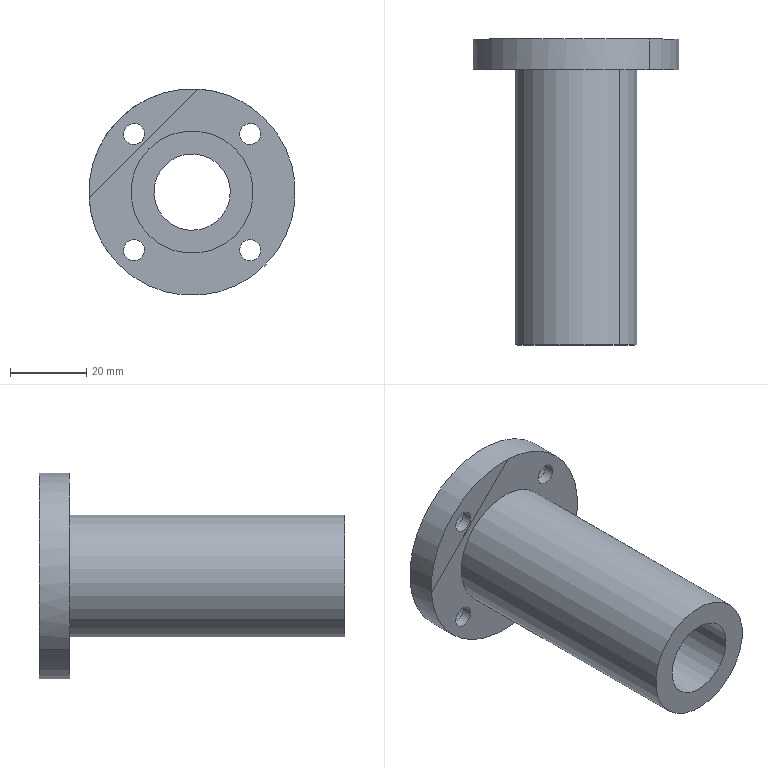Component | SolidWorks | LinearBearing20mmStandardRoundFlangeDoubleLinerTypeLMF20LUU-1 | 1 solid | 31 faces | box 54 x 80 x 54 mm | volume 49314 mm3 | cylinder 22 | plane 9 | commonest cylinder face diameters 9.5 x8 5.5 x8 20 x2 32 x2 54 x2
build123d program:
from build123d import *

# Parameters (mm, degrees)
SKETCH1_R                                       = 27
BOSS_EXTRUDE1_DEPTH                             = 8
SKETCH2_R                                       = 16
BOSS_EXTRUDE2_DEPTH                             = 72
SKETCH3_R                                       = 10
CUT_EXTRUDE1_DEPTH                              = 89.645
M5_HEX_SOCKET_HEAD_CAP_SCREW_CBORE1_D           = 5.5
M5_HEX_SOCKET_HEAD_CAP_SCREW_CBORE1_CBORE_D     = 9.5
M5_HEX_SOCKET_HEAD_CAP_SCREW_CBORE1_CBORE_DEPTH = 5.4
CIRPATTERN1_COUNT                               = 4
SKETCH7_W                                       = 60.924
SKETCH7_H                                       = 19.438
CUT_EXTRUDE2_DEPTH                              = 0.01


with BuildPart() as part:
    # Sketch1 → Boss-Extrude1 (new body)
    with BuildSketch(Plane.XY):
        Circle(SKETCH1_R)
    extrude(amount=BOSS_EXTRUDE1_DEPTH)

    # Sketch2 → Boss-Extrude2 (add)
    with BuildSketch(Plane.XY.offset(8)):
        Circle(SKETCH2_R)
    extrude(amount=BOSS_EXTRUDE2_DEPTH)

    # Sketch3 → Cut-Extrude1 (cut, through all)
    with BuildSketch(Plane(origin=(0, 0, 0), x_dir=(-1, 0, 0), z_dir=(0, 0, -1))):
        Circle(SKETCH3_R)
    extrude(amount=-CUT_EXTRUDE1_DEPTH, mode=Mode.SUBTRACT)

    # M5 Hex Socket Head Cap Screw CBORE1 (through all)
    with Locations(Plane(origin=(0, 0, 0), x_dir=(-1, 0, 0), z_dir=(0, 0, -1))):
        with Locations((0, -21.5)):
            m5_hex_socket_head_cap_screw_cbore1 = CounterBoreHole(M5_HEX_SOCKET_HEAD_CAP_SCREW_CBORE1_D / 2, M5_HEX_SOCKET_HEAD_CAP_SCREW_CBORE1_CBORE_D / 2, M5_HEX_SOCKET_HEAD_CAP_SCREW_CBORE1_CBORE_DEPTH)

    # CirPattern1: M5 Hex Socket Head Cap Screw CBORE1 ×4 about axis
    cirpattern1_axis = Axis((0, 0, 0), (0, 0, 1))
    for i in range(1, CIRPATTERN1_COUNT):
        add(m5_hex_socket_head_cap_screw_cbore1.rotate(cirpattern1_axis, i * 360 / CIRPATTERN1_COUNT), mode=Mode.SUBTRACT)

    # Sketch7 → Cut-Extrude2 (cut)
    with BuildSketch(Plane.XY.offset(8)):
        with Locations((-1.946, -27.719)):
            Rectangle(SKETCH7_W, SKETCH7_H)
    extrude(amount=-CUT_EXTRUDE2_DEPTH, mode=Mode.SUBTRACT)


solid = part.part

# Placed as in the assembly
solid = solid.moved(Location((-641.612, -154.873, 2398.4), (90, 0, -135)))
STEP:
#1=COLOUR_RGB('',0.7922,0.8196,0.9333);
#2=FILL_AREA_STYLE_COLOUR('',#1);
#3=FILL_AREA_STYLE('',(#2));
#4=SURFACE_STYLE_FILL_AREA(#3);
#5=SURFACE_SIDE_STYLE('',(#4));
#6=SURFACE_STYLE_USAGE(.BOTH.,#5);
#7=PRESENTATION_STYLE_ASSIGNMENT((#6));
#8=CARTESIAN_POINT('',(-25.991,-6.31,93.694));
#9=VERTEX_POINT('',#8);
#10=CARTESIAN_POINT('',(-25.727,-6.31,93.959));
#11=VERTEX_POINT('',#10);
#12=CARTESIAN_POINT('',(-25.859,-6.31,93.827));
#13=DIRECTION('',(-0.,1.,-0.));
#14=DIRECTION('',(0.7071,0.,0.7071));
#15=AXIS2_PLACEMENT_3D('',#12,#13,#14);
#16=CIRCLE('',#15,0.187);
#17=EDGE_CURVE('',#9,#11,#16,.T.);
#18=ORIENTED_EDGE('',*,*,#17,.F.);
#19=CARTESIAN_POINT('',(-25.991,-6.097,93.694));
#20=VERTEX_POINT('',#19);
#21=CARTESIAN_POINT('',(-25.991,-6.097,93.694));
#22=DIRECTION('',(-0.,1.,-0.));
#23=VECTOR('',#22,39.37);
#24=LINE('',#21,#23);
#25=EDGE_CURVE('',#9,#20,#24,.T.);
#26=ORIENTED_EDGE('',*,*,#25,.T.);
#27=CARTESIAN_POINT('',(-25.727,-6.097,93.959));
#28=VERTEX_POINT('',#27);
#29=CARTESIAN_POINT('',(-25.859,-6.097,93.827));
#30=DIRECTION('',(-0.,1.,-0.));
#31=DIRECTION('',(0.7071,0.,0.7071));
#32=AXIS2_PLACEMENT_3D('',#29,#30,#31);
#33=CIRCLE('',#32,0.187);
#34=EDGE_CURVE('',#20,#28,#33,.T.);
#35=ORIENTED_EDGE('',*,*,#34,.T.);
#36=CARTESIAN_POINT('',(-25.727,-6.097,93.959));
#37=DIRECTION('',(-0.,1.,-0.));
#38=VECTOR('',#37,39.37);
#39=LINE('',#36,#38);
#40=EDGE_CURVE('',#11,#28,#39,.T.);
#41=ORIENTED_EDGE('',*,*,#40,.F.);
#42=EDGE_LOOP('',(#18,#26,#35,#41));
#43=FACE_OUTER_BOUND('',#42,.T.);
#44=CARTESIAN_POINT('',(-25.859,-6.097,93.827));
#45=DIRECTION('',(-0.,1.,-0.));
#46=DIRECTION('',(0.7071,0.,0.7071));
#47=AXIS2_PLACEMENT_3D('',#44,#45,#46);
#48=CYLINDRICAL_SURFACE('',#47,0.187);
#49=ADVANCED_FACE('',(#43),#48,.F.);
#50=CARTESIAN_POINT('',(-25.782,-6.412,93.903));
#51=VERTEX_POINT('',#50);
#52=CARTESIAN_POINT('',(-25.935,-6.412,93.75));
#53=VERTEX_POINT('',#52);
#54=CARTESIAN_POINT('',(-25.859,-6.412,93.827));
#55=DIRECTION('',(0.,-1.,0.));
#56=DIRECTION('',(-0.7071,0.,-0.7071));
#57=AXIS2_PLACEMENT_3D('',#54,#55,#56);
#58=CIRCLE('',#57,0.1083);
#59=EDGE_CURVE('',#51,#53,#58,.T.);
#60=ORIENTED_EDGE('',*,*,#59,.T.);
#61=CARTESIAN_POINT('',(-25.935,-6.31,93.75));
#62=VERTEX_POINT('',#61);
#63=CARTESIAN_POINT('',(-25.935,-6.097,93.75));
#64=DIRECTION('',(-0.,1.,-0.));
#65=VECTOR('',#64,39.37);
#66=LINE('',#63,#65);
#67=EDGE_CURVE('',#53,#62,#66,.T.);
#68=ORIENTED_EDGE('',*,*,#67,.T.);
#69=CARTESIAN_POINT('',(-25.782,-6.31,93.903));
#70=VERTEX_POINT('',#69);
#71=CARTESIAN_POINT('',(-25.859,-6.31,93.827));
#72=DIRECTION('',(-0.,1.,-0.));
#73=DIRECTION('',(0.7071,0.,0.7071));
#74=AXIS2_PLACEMENT_3D('',#71,#72,#73);
#75=CIRCLE('',#74,0.1083);
#76=EDGE_CURVE('',#62,#70,#75,.T.);
#77=ORIENTED_EDGE('',*,*,#76,.T.);
#78=CARTESIAN_POINT('',(-25.782,-6.097,93.903));
#79=DIRECTION('',(-0.,1.,-0.));
#80=VECTOR('',#79,39.37);
#81=LINE('',#78,#80);
#82=EDGE_CURVE('',#51,#70,#81,.T.);
#83=ORIENTED_EDGE('',*,*,#82,.F.);
#84=EDGE_LOOP('',(#60,#68,#77,#83));
#85=FACE_OUTER_BOUND('',#84,.T.);
#86=CARTESIAN_POINT('',(-25.859,-6.097,93.827));
#87=DIRECTION('',(-0.,1.,-0.));
#88=DIRECTION('',(0.7071,0.,0.7071));
#89=AXIS2_PLACEMENT_3D('',#86,#87,#88);
#90=CYLINDRICAL_SURFACE('',#89,0.1083);
#91=ADVANCED_FACE('',(#85),#90,.F.);
#92=CARTESIAN_POINT('',(-24.794,-6.31,93.694));
#93=VERTEX_POINT('',#92);
#94=CARTESIAN_POINT('',(-24.53,-6.31,93.959));
#95=VERTEX_POINT('',#94);
#96=CARTESIAN_POINT('',(-24.662,-6.31,93.827));
#97=DIRECTION('',(-0.,1.,-0.));
#98=DIRECTION('',(0.7071,0.,0.7071));
#99=AXIS2_PLACEMENT_3D('',#96,#97,#98);
#100=CIRCLE('',#99,0.187);
#101=EDGE_CURVE('',#93,#95,#100,.T.);
#102=ORIENTED_EDGE('',*,*,#101,.F.);
#103=CARTESIAN_POINT('',(-24.794,-6.097,93.694));
#104=VERTEX_POINT('',#103);
#105=CARTESIAN_POINT('',(-24.794,-6.097,93.694));
#106=DIRECTION('',(-0.,1.,-0.));
#107=VECTOR('',#106,39.37);
#108=LINE('',#105,#107);
#109=EDGE_CURVE('',#93,#104,#108,.T.);
#110=ORIENTED_EDGE('',*,*,#109,.T.);
#111=CARTESIAN_POINT('',(-24.53,-6.097,93.959));
#112=VERTEX_POINT('',#111);
#113=CARTESIAN_POINT('',(-24.662,-6.097,93.827));
#114=DIRECTION('',(-0.,1.,-0.));
#115=DIRECTION('',(0.7071,0.,0.7071));
#116=AXIS2_PLACEMENT_3D('',#113,#114,#115);
#117=CIRCLE('',#116,0.187);
#118=EDGE_CURVE('',#104,#112,#117,.T.);
#119=ORIENTED_EDGE('',*,*,#118,.T.);
#120=CARTESIAN_POINT('',(-24.53,-6.097,93.959));
#121=DIRECTION('',(-0.,1.,-0.));
#122=VECTOR('',#121,39.37);
#123=LINE('',#120,#122);
#124=EDGE_CURVE('',#95,#112,#123,.T.);
#125=ORIENTED_EDGE('',*,*,#124,.F.);
#126=EDGE_LOOP('',(#102,#110,#119,#125));
#127=FACE_OUTER_BOUND('',#126,.T.);
#128=CARTESIAN_POINT('',(-24.662,-6.097,93.827));
#129=DIRECTION('',(-0.,1.,-0.));
#130=DIRECTION('',(0.7071,0.,0.7071));
#131=AXIS2_PLACEMENT_3D('',#128,#129,#130);
#132=CYLINDRICAL_SURFACE('',#131,0.187);
#133=ADVANCED_FACE('',(#127),#132,.F.);
#134=CARTESIAN_POINT('',(-24.585,-6.412,93.903));
#135=VERTEX_POINT('',#134);
#136=CARTESIAN_POINT('',(-24.738,-6.412,93.75));
#137=VERTEX_POINT('',#136);
#138=CARTESIAN_POINT('',(-24.662,-6.412,93.827));
#139=DIRECTION('',(0.,-1.,0.));
#140=DIRECTION('',(-0.7071,0.,-0.7071));
#141=AXIS2_PLACEMENT_3D('',#138,#139,#140);
#142=CIRCLE('',#141,0.1083);
#143=EDGE_CURVE('',#135,#137,#142,.T.);
#144=ORIENTED_EDGE('',*,*,#143,.T.);
#145=CARTESIAN_POINT('',(-24.738,-6.31,93.75));
#146=VERTEX_POINT('',#145);
#147=CARTESIAN_POINT('',(-24.738,-6.097,93.75));
#148=DIRECTION('',(-0.,1.,-0.));
#149=VECTOR('',#148,39.37);
#150=LINE('',#147,#149);
#151=EDGE_CURVE('',#137,#146,#150,.T.);
#152=ORIENTED_EDGE('',*,*,#151,.T.);
#153=CARTESIAN_POINT('',(-24.585,-6.31,93.903));
#154=VERTEX_POINT('',#153);
#155=CARTESIAN_POINT('',(-24.662,-6.31,93.827));
#156=DIRECTION('',(-0.,1.,-0.));
#157=DIRECTION('',(0.7071,0.,0.7071));
#158=AXIS2_PLACEMENT_3D('',#155,#156,#157);
#159=CIRCLE('',#158,0.1083);
#160=EDGE_CURVE('',#146,#154,#159,.T.);
#161=ORIENTED_EDGE('',*,*,#160,.T.);
#162=CARTESIAN_POINT('',(-24.585,-6.097,93.903));
#163=DIRECTION('',(-0.,1.,-0.));
#164=VECTOR('',#163,39.37);
#165=LINE('',#162,#164);
#166=EDGE_CURVE('',#135,#154,#165,.T.);
#167=ORIENTED_EDGE('',*,*,#166,.F.);
#168=EDGE_LOOP('',(#144,#152,#161,#167));
#169=FACE_OUTER_BOUND('',#168,.T.);
#170=CARTESIAN_POINT('',(-24.662,-6.097,93.827));
#171=DIRECTION('',(-0.,1.,-0.));
#172=DIRECTION('',(0.7071,0.,0.7071));
#173=AXIS2_PLACEMENT_3D('',#170,#171,#172);
#174=CYLINDRICAL_SURFACE('',#173,0.1083);
#175=ADVANCED_FACE('',(#169),#174,.F.);
#176=CARTESIAN_POINT('',(-24.794,-6.31,94.891));
#177=VERTEX_POINT('',#176);
#178=CARTESIAN_POINT('',(-24.53,-6.31,95.156));
#179=VERTEX_POINT('',#178);
#180=CARTESIAN_POINT('',(-24.662,-6.31,95.024));
#181=DIRECTION('',(-0.,1.,-0.));
#182=DIRECTION('',(0.7071,0.,0.7071));
#183=AXIS2_PLACEMENT_3D('',#180,#181,#182);
#184=CIRCLE('',#183,0.187);
#185=EDGE_CURVE('',#177,#179,#184,.T.);
#186=ORIENTED_EDGE('',*,*,#185,.F.);
#187=CARTESIAN_POINT('',(-24.794,-6.097,94.891));
#188=VERTEX_POINT('',#187);
#189=CARTESIAN_POINT('',(-24.794,-6.097,94.891));
#190=DIRECTION('',(-0.,1.,-0.));
#191=VECTOR('',#190,39.37);
#192=LINE('',#189,#191);
#193=EDGE_CURVE('',#177,#188,#192,.T.);
#194=ORIENTED_EDGE('',*,*,#193,.T.);
#195=CARTESIAN_POINT('',(-24.53,-6.097,95.156));
#196=VERTEX_POINT('',#195);
#197=CARTESIAN_POINT('',(-24.662,-6.097,95.024));
#198=DIRECTION('',(-0.,1.,-0.));
#199=DIRECTION('',(0.7071,0.,0.7071));
#200=AXIS2_PLACEMENT_3D('',#197,#198,#199);
#201=CIRCLE('',#200,0.187);
#202=EDGE_CURVE('',#188,#196,#201,.T.);
#203=ORIENTED_EDGE('',*,*,#202,.T.);
#204=CARTESIAN_POINT('',(-24.53,-6.097,95.156));
#205=DIRECTION('',(-0.,1.,-0.));
#206=VECTOR('',#205,39.37);
#207=LINE('',#204,#206);
#208=EDGE_CURVE('',#179,#196,#207,.T.);
#209=ORIENTED_EDGE('',*,*,#208,.F.);
#210=EDGE_LOOP('',(#186,#194,#203,#209));
#211=FACE_OUTER_BOUND('',#210,.T.);
#212=CARTESIAN_POINT('',(-24.662,-6.097,95.024));
#213=DIRECTION('',(-0.,1.,-0.));
#214=DIRECTION('',(0.7071,0.,0.7071));
#215=AXIS2_PLACEMENT_3D('',#212,#213,#214);
#216=CYLINDRICAL_SURFACE('',#215,0.187);
#217=ADVANCED_FACE('',(#211),#216,.F.);
#218=CARTESIAN_POINT('',(-24.585,-6.412,95.1));
#219=VERTEX_POINT('',#218);
#220=CARTESIAN_POINT('',(-24.738,-6.412,94.947));
#221=VERTEX_POINT('',#220);
#222=CARTESIAN_POINT('',(-24.662,-6.412,95.024));
#223=DIRECTION('',(0.,-1.,0.));
#224=DIRECTION('',(-0.7071,0.,-0.7071));
#225=AXIS2_PLACEMENT_3D('',#222,#223,#224);
#226=CIRCLE('',#225,0.1083);
#227=EDGE_CURVE('',#219,#221,#226,.T.);
#228=ORIENTED_EDGE('',*,*,#227,.T.);
#229=CARTESIAN_POINT('',(-24.738,-6.31,94.947));
#230=VERTEX_POINT('',#229);
#231=CARTESIAN_POINT('',(-24.738,-6.097,94.947));
#232=DIRECTION('',(-0.,1.,-0.));
#233=VECTOR('',#232,39.37);
#234=LINE('',#231,#233);
#235=EDGE_CURVE('',#221,#230,#234,.T.);
#236=ORIENTED_EDGE('',*,*,#235,.T.);
#237=CARTESIAN_POINT('',(-24.585,-6.31,95.1));
#238=VERTEX_POINT('',#237);
#239=CARTESIAN_POINT('',(-24.662,-6.31,95.024));
#240=DIRECTION('',(-0.,1.,-0.));
#241=DIRECTION('',(0.7071,0.,0.7071));
#242=AXIS2_PLACEMENT_3D('',#239,#240,#241);
#243=CIRCLE('',#242,0.1083);
#244=EDGE_CURVE('',#230,#238,#243,.T.);
#245=ORIENTED_EDGE('',*,*,#244,.T.);
#246=CARTESIAN_POINT('',(-24.585,-6.097,95.1));
#247=DIRECTION('',(-0.,1.,-0.));
#248=VECTOR('',#247,39.37);
#249=LINE('',#246,#248);
#250=EDGE_CURVE('',#219,#238,#249,.T.);
#251=ORIENTED_EDGE('',*,*,#250,.F.);
#252=EDGE_LOOP('',(#228,#236,#245,#251));
#253=FACE_OUTER_BOUND('',#252,.T.);
#254=CARTESIAN_POINT('',(-24.662,-6.097,95.024));
#255=DIRECTION('',(-0.,1.,-0.));
#256=DIRECTION('',(0.7071,0.,0.7071));
#257=AXIS2_PLACEMENT_3D('',#254,#255,#256);
#258=CYLINDRICAL_SURFACE('',#257,0.1083);
#259=ADVANCED_FACE('',(#253),#258,.F.);
#260=CARTESIAN_POINT('',(-25.991,-6.31,94.891));
#261=VERTEX_POINT('',#260);
#262=CARTESIAN_POINT('',(-25.727,-6.31,95.156));
#263=VERTEX_POINT('',#262);
#264=CARTESIAN_POINT('',(-25.859,-6.31,95.024));
#265=DIRECTION('',(-0.,1.,-0.));
#266=DIRECTION('',(0.7071,0.,0.7071));
#267=AXIS2_PLACEMENT_3D('',#264,#265,#266);
#268=CIRCLE('',#267,0.187);
#269=EDGE_CURVE('',#261,#263,#268,.T.);
#270=ORIENTED_EDGE('',*,*,#269,.F.);
#271=CARTESIAN_POINT('',(-25.991,-6.097,94.891));
#272=VERTEX_POINT('',#271);
#273=CARTESIAN_POINT('',(-25.991,-6.097,94.891));
#274=DIRECTION('',(-0.,1.,-0.));
#275=VECTOR('',#274,39.37);
#276=LINE('',#273,#275);
#277=EDGE_CURVE('',#261,#272,#276,.T.);
#278=ORIENTED_EDGE('',*,*,#277,.T.);
#279=CARTESIAN_POINT('',(-25.727,-6.097,95.156));
#280=VERTEX_POINT('',#279);
#281=CARTESIAN_POINT('',(-25.859,-6.097,95.024));
#282=DIRECTION('',(-0.,1.,-0.));
#283=DIRECTION('',(0.7071,0.,0.7071));
#284=AXIS2_PLACEMENT_3D('',#281,#282,#283);
#285=CIRCLE('',#284,0.187);
#286=EDGE_CURVE('',#272,#280,#285,.T.);
#287=ORIENTED_EDGE('',*,*,#286,.T.);
#288=CARTESIAN_POINT('',(-25.727,-6.097,95.156));
#289=DIRECTION('',(-0.,1.,-0.));
#290=VECTOR('',#289,39.37);
#291=LINE('',#288,#290);
#292=EDGE_CURVE('',#263,#280,#291,.T.);
#293=ORIENTED_EDGE('',*,*,#292,.F.);
#294=EDGE_LOOP('',(#270,#278,#287,#293));
#295=FACE_OUTER_BOUND('',#294,.T.);
#296=CARTESIAN_POINT('',(-25.859,-6.097,95.024));
#297=DIRECTION('',(-0.,1.,-0.));
#298=DIRECTION('',(0.7071,0.,0.7071));
#299=AXIS2_PLACEMENT_3D('',#296,#297,#298);
#300=CYLINDRICAL_SURFACE('',#299,0.187);
#301=ADVANCED_FACE('',(#295),#300,.F.);
#302=CARTESIAN_POINT('',(-25.539,-9.247,94.147));
#303=VERTEX_POINT('',#302);
#304=CARTESIAN_POINT('',(-24.982,-9.247,94.704));
#305=VERTEX_POINT('',#304);
#306=CARTESIAN_POINT('',(-25.26,-9.247,94.425));
#307=DIRECTION('',(-0.,1.,-0.));
#308=DIRECTION('',(0.7071,0.,0.7071));
#309=AXIS2_PLACEMENT_3D('',#306,#307,#308);
#310=CIRCLE('',#309,0.3937);
#311=EDGE_CURVE('',#303,#305,#310,.T.);
#312=ORIENTED_EDGE('',*,*,#311,.F.);
#313=CARTESIAN_POINT('',(-25.539,-6.097,94.147));
#314=VERTEX_POINT('',#313);
#315=CARTESIAN_POINT('',(-25.539,-9.247,94.147));
#316=DIRECTION('',(-0.,1.,-0.));
#317=VECTOR('',#316,39.37);
#318=LINE('',#315,#317);
#319=EDGE_CURVE('',#303,#314,#318,.T.);
#320=ORIENTED_EDGE('',*,*,#319,.T.);
#321=CARTESIAN_POINT('',(-24.982,-6.097,94.704));
#322=VERTEX_POINT('',#321);
#323=CARTESIAN_POINT('',(-25.26,-6.097,94.425));
#324=DIRECTION('',(-0.,1.,-0.));
#325=DIRECTION('',(0.7071,0.,0.7071));
#326=AXIS2_PLACEMENT_3D('',#323,#324,#325);
#327=CIRCLE('',#326,0.3937);
#328=EDGE_CURVE('',#314,#322,#327,.T.);
#329=ORIENTED_EDGE('',*,*,#328,.T.);
#330=CARTESIAN_POINT('',(-24.982,-9.247,94.704));
#331=DIRECTION('',(-0.,1.,-0.));
#332=VECTOR('',#331,39.37);
#333=LINE('',#330,#332);
#334=EDGE_CURVE('',#305,#322,#333,.T.);
#335=ORIENTED_EDGE('',*,*,#334,.F.);
#336=EDGE_LOOP('',(#312,#320,#329,#335));
#337=FACE_OUTER_BOUND('',#336,.T.);
#338=CARTESIAN_POINT('',(-25.26,-9.247,94.425));
#339=DIRECTION('',(-0.,1.,-0.));
#340=DIRECTION('',(0.7071,0.,0.7071));
#341=AXIS2_PLACEMENT_3D('',#338,#339,#340);
#342=CYLINDRICAL_SURFACE('',#341,0.3937);
#343=ADVANCED_FACE('',(#337),#342,.F.);
#344=CARTESIAN_POINT('',(-25.706,-9.247,93.98));
#345=VERTEX_POINT('',#344);
#346=CARTESIAN_POINT('',(-24.815,-9.247,94.871));
#347=VERTEX_POINT('',#346);
#348=CARTESIAN_POINT('',(-25.26,-9.247,94.425));
#349=DIRECTION('',(0.,-1.,0.));
#350=DIRECTION('',(-0.7071,0.,-0.7071));
#351=AXIS2_PLACEMENT_3D('',#348,#349,#350);
#352=CIRCLE('',#351,0.6299);
#353=EDGE_CURVE('',#345,#347,#352,.T.);
#354=ORIENTED_EDGE('',*,*,#353,.F.);
#355=CARTESIAN_POINT('',(-25.706,-6.412,93.98));
#356=VERTEX_POINT('',#355);
#357=CARTESIAN_POINT('',(-25.706,-9.247,93.98));
#358=DIRECTION('',(-0.,1.,-0.));
#359=VECTOR('',#358,39.37);
#360=LINE('',#357,#359);
#361=EDGE_CURVE('',#345,#356,#360,.T.);
#362=ORIENTED_EDGE('',*,*,#361,.T.);
#363=CARTESIAN_POINT('',(-24.815,-6.412,94.871));
#364=VERTEX_POINT('',#363);
#365=CARTESIAN_POINT('',(-25.26,-6.412,94.425));
#366=DIRECTION('',(0.,-1.,0.));
#367=DIRECTION('',(-0.7071,0.,-0.7071));
#368=AXIS2_PLACEMENT_3D('',#365,#366,#367);
#369=CIRCLE('',#368,0.6299);
#370=EDGE_CURVE('',#356,#364,#369,.T.);
#371=ORIENTED_EDGE('',*,*,#370,.T.);
#372=CARTESIAN_POINT('',(-24.815,-9.247,94.871));
#373=DIRECTION('',(-0.,1.,-0.));
#374=VECTOR('',#373,39.37);
#375=LINE('',#372,#374);
#376=EDGE_CURVE('',#347,#364,#375,.T.);
#377=ORIENTED_EDGE('',*,*,#376,.F.);
#378=EDGE_LOOP('',(#354,#362,#371,#377));
#379=FACE_OUTER_BOUND('',#378,.T.);
#380=CARTESIAN_POINT('',(-25.26,-9.247,94.425));
#381=DIRECTION('',(-0.,1.,-0.));
#382=DIRECTION('',(0.7071,0.,0.7071));
#383=AXIS2_PLACEMENT_3D('',#380,#381,#382);
#384=CYLINDRICAL_SURFACE('',#383,0.6299);
#385=ADVANCED_FACE('',(#379),#384,.T.);
#386=CARTESIAN_POINT('',(-26.012,-6.412,93.674));
#387=VERTEX_POINT('',#386);
#388=CARTESIAN_POINT('',(-24.509,-6.412,95.177));
#389=VERTEX_POINT('',#388);
#390=CARTESIAN_POINT('',(-25.26,-6.412,94.425));
#391=DIRECTION('',(0.,-1.,0.));
#392=DIRECTION('',(-0.7071,0.,-0.7071));
#393=AXIS2_PLACEMENT_3D('',#390,#391,#392);
#394=CIRCLE('',#393,1.063);
#395=EDGE_CURVE('',#387,#389,#394,.T.);
#396=ORIENTED_EDGE('',*,*,#395,.F.);
#397=CARTESIAN_POINT('',(-26.012,-6.097,93.674));
#398=VERTEX_POINT('',#397);
#399=CARTESIAN_POINT('',(-26.012,-6.412,93.674));
#400=DIRECTION('',(-0.,1.,-0.));
#401=VECTOR('',#400,39.37);
#402=LINE('',#399,#401);
#403=EDGE_CURVE('',#387,#398,#402,.T.);
#404=ORIENTED_EDGE('',*,*,#403,.T.);
#405=CARTESIAN_POINT('',(-24.509,-6.097,95.177));
#406=VERTEX_POINT('',#405);
#407=CARTESIAN_POINT('',(-25.26,-6.097,94.425));
#408=DIRECTION('',(0.,-1.,0.));
#409=DIRECTION('',(-0.7071,0.,-0.7071));
#410=AXIS2_PLACEMENT_3D('',#407,#408,#409);
#411=CIRCLE('',#410,1.063);
#412=EDGE_CURVE('',#398,#406,#411,.T.);
#413=ORIENTED_EDGE('',*,*,#412,.T.);
#414=CARTESIAN_POINT('',(-24.509,-6.412,95.177));
#415=DIRECTION('',(-0.,1.,-0.));
#416=VECTOR('',#415,39.37);
#417=LINE('',#414,#416);
#418=EDGE_CURVE('',#389,#406,#417,.T.);
#419=ORIENTED_EDGE('',*,*,#418,.F.);
#420=EDGE_LOOP('',(#396,#404,#413,#419));
#421=FACE_OUTER_BOUND('',#420,.T.);
#422=CARTESIAN_POINT('',(-25.26,-6.412,94.425));
#423=DIRECTION('',(-0.,1.,-0.));
#424=DIRECTION('',(0.7071,0.,0.7071));
#425=AXIS2_PLACEMENT_3D('',#422,#423,#424);
#426=CYLINDRICAL_SURFACE('',#425,1.063);
#427=ADVANCED_FACE('',(#421),#426,.T.);
#428=CARTESIAN_POINT('',(-25.935,-6.412,94.947));
#429=VERTEX_POINT('',#428);
#430=CARTESIAN_POINT('',(-25.782,-6.412,95.1));
#431=VERTEX_POINT('',#430);
#432=CARTESIAN_POINT('',(-25.859,-6.412,95.024));
#433=DIRECTION('',(-0.,1.,-0.));
#434=DIRECTION('',(-0.7071,0.,-0.7071));
#435=AXIS2_PLACEMENT_3D('',#432,#433,#434);
#436=CIRCLE('',#435,0.1083);
#437=EDGE_CURVE('',#429,#431,#436,.T.);
#438=ORIENTED_EDGE('',*,*,#437,.F.);
#439=CARTESIAN_POINT('',(-25.935,-6.31,94.947));
#440=VERTEX_POINT('',#439);
#441=CARTESIAN_POINT('',(-25.935,-6.097,94.947));
#442=DIRECTION('',(-0.,1.,-0.));
#443=VECTOR('',#442,39.37);
#444=LINE('',#441,#443);
#445=EDGE_CURVE('',#429,#440,#444,.T.);
#446=ORIENTED_EDGE('',*,*,#445,.T.);
#447=CARTESIAN_POINT('',(-25.782,-6.31,95.1));
#448=VERTEX_POINT('',#447);
#449=CARTESIAN_POINT('',(-25.859,-6.31,95.024));
#450=DIRECTION('',(-0.,1.,-0.));
#451=DIRECTION('',(0.7071,0.,0.7071));
#452=AXIS2_PLACEMENT_3D('',#449,#450,#451);
#453=CIRCLE('',#452,0.1083);
#454=EDGE_CURVE('',#440,#448,#453,.T.);
#455=ORIENTED_EDGE('',*,*,#454,.T.);
#456=CARTESIAN_POINT('',(-25.782,-6.097,95.1));
#457=DIRECTION('',(-0.,1.,-0.));
#458=VECTOR('',#457,39.37);
#459=LINE('',#456,#458);
#460=EDGE_CURVE('',#431,#448,#459,.T.);
#461=ORIENTED_EDGE('',*,*,#460,.F.);
#462=EDGE_LOOP('',(#438,#446,#455,#461));
#463=FACE_OUTER_BOUND('',#462,.T.);
#464=CARTESIAN_POINT('',(-25.859,-6.097,95.024));
#465=DIRECTION('',(-0.,1.,-0.));
#466=DIRECTION('',(0.7071,0.,0.7071));
#467=AXIS2_PLACEMENT_3D('',#464,#465,#466);
#468=CYLINDRICAL_SURFACE('',#467,0.1083);
#469=ADVANCED_FACE('',(#463),#468,.F.);
#470=ORIENTED_EDGE('',*,*,#445,.F.);
#471=CARTESIAN_POINT('',(-25.859,-6.412,95.024));
#472=DIRECTION('',(-0.,1.,-0.));
#473=DIRECTION('',(-0.7071,0.,-0.7071));
#474=AXIS2_PLACEMENT_3D('',#471,#472,#473);
#475=CIRCLE('',#474,0.1083);
#476=EDGE_CURVE('',#431,#429,#475,.T.);
#477=ORIENTED_EDGE('',*,*,#476,.F.);
#478=ORIENTED_EDGE('',*,*,#460,.T.);
#479=CARTESIAN_POINT('',(-25.859,-6.31,95.024));
#480=DIRECTION('',(-0.,1.,-0.));
#481=DIRECTION('',(0.7071,0.,0.7071));
#482=AXIS2_PLACEMENT_3D('',#479,#480,#481);
#483=CIRCLE('',#482,0.1083);
#484=EDGE_CURVE('',#448,#440,#483,.T.);
#485=ORIENTED_EDGE('',*,*,#484,.T.);
#486=EDGE_LOOP('',(#470,#477,#478,#485));
#487=FACE_OUTER_BOUND('',#486,.T.);
#488=CARTESIAN_POINT('',(-25.859,-6.097,95.024));
#489=DIRECTION('',(-0.,1.,-0.));
#490=DIRECTION('',(0.7071,0.,0.7071));
#491=AXIS2_PLACEMENT_3D('',#488,#489,#490);
#492=CYLINDRICAL_SURFACE('',#491,0.1083);
#493=ADVANCED_FACE('',(#487),#492,.F.);
#494=CARTESIAN_POINT('',(-26.322,-6.412,94.366));
#495=VERTEX_POINT('',#494);
#496=CARTESIAN_POINT('',(-25.201,-6.412,95.487));
#497=VERTEX_POINT('',#496);
#498=CARTESIAN_POINT('',(-26.555,-6.412,94.132));
#499=DIRECTION('',(0.7071,0.,0.7071));
#500=VECTOR('',#499,39.37);
#501=LINE('',#498,#500);
#502=EDGE_CURVE('',#495,#497,#501,.T.);
#503=ORIENTED_EDGE('',*,*,#502,.F.);
#504=CARTESIAN_POINT('',(-25.26,-6.412,94.425));
#505=DIRECTION('',(0.,-1.,0.));
#506=DIRECTION('',(-0.7071,0.,-0.7071));
#507=AXIS2_PLACEMENT_3D('',#504,#505,#506);
#508=CIRCLE('',#507,1.063);
#509=EDGE_CURVE('',#495,#387,#508,.T.);
#510=ORIENTED_EDGE('',*,*,#509,.T.);
#511=ORIENTED_EDGE('',*,*,#395,.T.);
#512=CARTESIAN_POINT('',(-25.26,-6.412,94.425));
#513=DIRECTION('',(0.,-1.,0.));
#514=DIRECTION('',(-0.7071,0.,-0.7071));
#515=AXIS2_PLACEMENT_3D('',#512,#513,#514);
#516=CIRCLE('',#515,1.063);
#517=EDGE_CURVE('',#389,#497,#516,.T.);
#518=ORIENTED_EDGE('',*,*,#517,.T.);
#519=EDGE_LOOP('',(#503,#510,#511,#518));
#520=FACE_OUTER_BOUND('',#519,.T.);
#521=ORIENTED_EDGE('',*,*,#59,.F.);
#522=CARTESIAN_POINT('',(-25.859,-6.412,93.827));
#523=DIRECTION('',(0.,-1.,0.));
#524=DIRECTION('',(-0.7071,0.,-0.7071));
#525=AXIS2_PLACEMENT_3D('',#522,#523,#524);
#526=CIRCLE('',#525,0.1083);
#527=EDGE_CURVE('',#53,#51,#526,.T.);
#528=ORIENTED_EDGE('',*,*,#527,.F.);
#529=EDGE_LOOP('',(#521,#528));
#530=FACE_BOUND('',#529,.T.);
#531=ORIENTED_EDGE('',*,*,#143,.F.);
#532=CARTESIAN_POINT('',(-24.662,-6.412,93.827));
#533=DIRECTION('',(0.,-1.,0.));
#534=DIRECTION('',(-0.7071,0.,-0.7071));
#535=AXIS2_PLACEMENT_3D('',#532,#533,#534);
#536=CIRCLE('',#535,0.1083);
#537=EDGE_CURVE('',#137,#135,#536,.T.);
#538=ORIENTED_EDGE('',*,*,#537,.F.);
#539=EDGE_LOOP('',(#531,#538));
#540=FACE_BOUND('',#539,.T.);
#541=ORIENTED_EDGE('',*,*,#227,.F.);
#542=CARTESIAN_POINT('',(-24.662,-6.412,95.024));
#543=DIRECTION('',(0.,-1.,0.));
#544=DIRECTION('',(-0.7071,0.,-0.7071));
#545=AXIS2_PLACEMENT_3D('',#542,#543,#544);
#546=CIRCLE('',#545,0.1083);
#547=EDGE_CURVE('',#221,#219,#546,.T.);
#548=ORIENTED_EDGE('',*,*,#547,.F.);
#549=EDGE_LOOP('',(#541,#548));
#550=FACE_BOUND('',#549,.T.);
#551=CARTESIAN_POINT('',(-25.26,-6.412,94.425));
#552=DIRECTION('',(0.,-1.,0.));
#553=DIRECTION('',(-0.7071,0.,-0.7071));
#554=AXIS2_PLACEMENT_3D('',#551,#552,#553);
#555=CIRCLE('',#554,0.6299);
#556=EDGE_CURVE('',#364,#356,#555,.T.);
#557=ORIENTED_EDGE('',*,*,#556,.F.);
#558=ORIENTED_EDGE('',*,*,#370,.F.);
#559=EDGE_LOOP('',(#557,#558));
#560=FACE_BOUND('',#559,.T.);
#561=CARTESIAN_POINT('',(-25.26,-6.412,94.425));
#562=DIRECTION('',(0.,-1.,0.));
#563=DIRECTION('',(-0.7071,-0.,-0.7071));
#564=AXIS2_PLACEMENT_3D('',#561,#562,#563);
#565=PLANE('',#564);
#566=ADVANCED_FACE('',(#520,#530,#540,#550,#560),#565,.T.);
#567=ORIENTED_EDGE('',*,*,#403,.F.);
#568=ORIENTED_EDGE('',*,*,#509,.F.);
#569=CARTESIAN_POINT('',(-26.322,-6.412,94.366));
#570=VERTEX_POINT('',#569);
#571=CARTESIAN_POINT('',(-26.322,-6.412,94.366));
#572=DIRECTION('',(-0.,1.,-0.));
#573=VECTOR('',#572,39.37);
#574=LINE('',#571,#573);
#575=EDGE_CURVE('',#495,#570,#574,.T.);
#576=ORIENTED_EDGE('',*,*,#575,.T.);
#577=CARTESIAN_POINT('',(-25.201,-6.412,95.487));
#578=VERTEX_POINT('',#577);
#579=CARTESIAN_POINT('',(-25.26,-6.412,94.425));
#580=DIRECTION('',(0.,-1.,0.));
#581=DIRECTION('',(-0.7071,0.,-0.7071));
#582=AXIS2_PLACEMENT_3D('',#579,#580,#581);
#583=CIRCLE('',#582,1.063);
#584=EDGE_CURVE('',#578,#570,#583,.T.);
#585=ORIENTED_EDGE('',*,*,#584,.F.);
#586=CARTESIAN_POINT('',(-25.201,-6.412,95.487));
#587=DIRECTION('',(0.,-1.,0.));
#588=VECTOR('',#587,39.37);
#589=LINE('',#586,#588);
#590=EDGE_CURVE('',#578,#497,#589,.T.);
#591=ORIENTED_EDGE('',*,*,#590,.T.);
#592=ORIENTED_EDGE('',*,*,#517,.F.);
#593=ORIENTED_EDGE('',*,*,#418,.T.);
#594=CARTESIAN_POINT('',(-25.26,-6.097,94.425));
#595=DIRECTION('',(0.,-1.,0.));
#596=DIRECTION('',(-0.7071,0.,-0.7071));
#597=AXIS2_PLACEMENT_3D('',#594,#595,#596);
#598=CIRCLE('',#597,1.063);
#599=EDGE_CURVE('',#406,#398,#598,.T.);
#600=ORIENTED_EDGE('',*,*,#599,.T.);
#601=EDGE_LOOP('',(#567,#568,#576,#585,#591,#592,#593,#600));
#602=FACE_OUTER_BOUND('',#601,.T.);
#603=CARTESIAN_POINT('',(-25.26,-6.412,94.425));
#604=DIRECTION('',(-0.,1.,-0.));
#605=DIRECTION('',(0.7071,0.,0.7071));
#606=AXIS2_PLACEMENT_3D('',#603,#604,#605);
#607=CYLINDRICAL_SURFACE('',#606,1.063);
#608=ADVANCED_FACE('',(#602),#607,.T.);
#609=CARTESIAN_POINT('',(-25.859,-6.097,93.827));
#610=DIRECTION('',(-0.,1.,-0.));
#611=DIRECTION('',(0.7071,0.,0.7071));
#612=AXIS2_PLACEMENT_3D('',#609,#610,#611);
#613=CIRCLE('',#612,0.187);
#614=EDGE_CURVE('',#28,#20,#613,.T.);
#615=ORIENTED_EDGE('',*,*,#614,.F.);
#616=ORIENTED_EDGE('',*,*,#34,.F.);
#617=EDGE_LOOP('',(#615,#616));
#618=FACE_BOUND('',#617,.T.);
#619=CARTESIAN_POINT('',(-24.662,-6.097,93.827));
#620=DIRECTION('',(-0.,1.,-0.));
#621=DIRECTION('',(0.7071,0.,0.7071));
#622=AXIS2_PLACEMENT_3D('',#619,#620,#621);
#623=CIRCLE('',#622,0.187);
#624=EDGE_CURVE('',#112,#104,#623,.T.);
#625=ORIENTED_EDGE('',*,*,#624,.F.);
#626=ORIENTED_EDGE('',*,*,#118,.F.);
#627=EDGE_LOOP('',(#625,#626));
#628=FACE_BOUND('',#627,.T.);
#629=CARTESIAN_POINT('',(-24.662,-6.097,95.024));
#630=DIRECTION('',(-0.,1.,-0.));
#631=DIRECTION('',(0.7071,0.,0.7071));
#632=AXIS2_PLACEMENT_3D('',#629,#630,#631);
#633=CIRCLE('',#632,0.187);
#634=EDGE_CURVE('',#196,#188,#633,.T.);
#635=ORIENTED_EDGE('',*,*,#634,.F.);
#636=ORIENTED_EDGE('',*,*,#202,.F.);
#637=EDGE_LOOP('',(#635,#636));
#638=FACE_BOUND('',#637,.T.);
#639=CARTESIAN_POINT('',(-25.859,-6.097,95.024));
#640=DIRECTION('',(-0.,1.,-0.));
#641=DIRECTION('',(0.7071,0.,0.7071));
#642=AXIS2_PLACEMENT_3D('',#639,#640,#641);
#643=CIRCLE('',#642,0.187);
#644=EDGE_CURVE('',#280,#272,#643,.T.);
#645=ORIENTED_EDGE('',*,*,#644,.F.);
#646=ORIENTED_EDGE('',*,*,#286,.F.);
#647=EDGE_LOOP('',(#645,#646));
#648=FACE_BOUND('',#647,.T.);
#649=CARTESIAN_POINT('',(-25.26,-6.097,94.425));
#650=DIRECTION('',(-0.,1.,-0.));
#651=DIRECTION('',(0.7071,0.,0.7071));
#652=AXIS2_PLACEMENT_3D('',#649,#650,#651);
#653=CIRCLE('',#652,0.3937);
#654=EDGE_CURVE('',#322,#314,#653,.T.);
#655=ORIENTED_EDGE('',*,*,#654,.F.);
#656=ORIENTED_EDGE('',*,*,#328,.F.);
#657=EDGE_LOOP('',(#655,#656));
#658=FACE_BOUND('',#657,.T.);
#659=ORIENTED_EDGE('',*,*,#599,.F.);
#660=ORIENTED_EDGE('',*,*,#412,.F.);
#661=EDGE_LOOP('',(#659,#660));
#662=FACE_OUTER_BOUND('',#661,.T.);
#663=CARTESIAN_POINT('',(-25.26,-6.097,94.425));
#664=DIRECTION('',(0.,-1.,0.));
#665=DIRECTION('',(-0.7071,-0.,-0.7071));
#666=AXIS2_PLACEMENT_3D('',#663,#664,#665);
#667=PLANE('',#666);
#668=ADVANCED_FACE('',(#618,#628,#638,#648,#658,#662),#667,.F.);
#669=ORIENTED_EDGE('',*,*,#361,.F.);
#670=CARTESIAN_POINT('',(-25.26,-9.247,94.425));
#671=DIRECTION('',(0.,-1.,0.));
#672=DIRECTION('',(-0.7071,0.,-0.7071));
#673=AXIS2_PLACEMENT_3D('',#670,#671,#672);
#674=CIRCLE('',#673,0.6299);
#675=EDGE_CURVE('',#347,#345,#674,.T.);
#676=ORIENTED_EDGE('',*,*,#675,.F.);
#677=ORIENTED_EDGE('',*,*,#376,.T.);
#678=ORIENTED_EDGE('',*,*,#556,.T.);
#679=EDGE_LOOP('',(#669,#676,#677,#678));
#680=FACE_OUTER_BOUND('',#679,.T.);
#681=CARTESIAN_POINT('',(-25.26,-9.247,94.425));
#682=DIRECTION('',(-0.,1.,-0.));
#683=DIRECTION('',(0.7071,0.,0.7071));
#684=AXIS2_PLACEMENT_3D('',#681,#682,#683);
#685=CYLINDRICAL_SURFACE('',#684,0.6299);
#686=ADVANCED_FACE('',(#680),#685,.T.);
#687=CARTESIAN_POINT('',(-25.26,-9.247,94.425));
#688=DIRECTION('',(-0.,1.,-0.));
#689=DIRECTION('',(0.7071,0.,0.7071));
#690=AXIS2_PLACEMENT_3D('',#687,#688,#689);
#691=CIRCLE('',#690,0.3937);
#692=EDGE_CURVE('',#305,#303,#691,.T.);
#693=ORIENTED_EDGE('',*,*,#692,.T.);
#694=ORIENTED_EDGE('',*,*,#311,.T.);
#695=EDGE_LOOP('',(#693,#694));
#696=FACE_BOUND('',#695,.T.);
#697=ORIENTED_EDGE('',*,*,#675,.T.);
#698=ORIENTED_EDGE('',*,*,#353,.T.);
#699=EDGE_LOOP('',(#697,#698));
#700=FACE_OUTER_BOUND('',#699,.T.);
#701=CARTESIAN_POINT('',(-25.26,-9.247,94.425));
#702=DIRECTION('',(0.,-1.,0.));
#703=DIRECTION('',(-0.7071,-0.,-0.7071));
#704=AXIS2_PLACEMENT_3D('',#701,#702,#703);
#705=PLANE('',#704);
#706=ADVANCED_FACE('',(#696,#700),#705,.T.);
#707=ORIENTED_EDGE('',*,*,#319,.F.);
#708=ORIENTED_EDGE('',*,*,#692,.F.);
#709=ORIENTED_EDGE('',*,*,#334,.T.);
#710=ORIENTED_EDGE('',*,*,#654,.T.);
#711=EDGE_LOOP('',(#707,#708,#709,#710));
#712=FACE_OUTER_BOUND('',#711,.T.);
#713=CARTESIAN_POINT('',(-25.26,-9.247,94.425));
#714=DIRECTION('',(-0.,1.,-0.));
#715=DIRECTION('',(0.7071,0.,0.7071));
#716=AXIS2_PLACEMENT_3D('',#713,#714,#715);
#717=CYLINDRICAL_SURFACE('',#716,0.3937);
#718=ADVANCED_FACE('',(#712),#717,.F.);
#719=ORIENTED_EDGE('',*,*,#484,.F.);
#720=ORIENTED_EDGE('',*,*,#454,.F.);
#721=EDGE_LOOP('',(#719,#720));
#722=FACE_BOUND('',#721,.T.);
#723=CARTESIAN_POINT('',(-25.859,-6.31,95.024));
#724=DIRECTION('',(-0.,1.,-0.));
#725=DIRECTION('',(0.7071,0.,0.7071));
#726=AXIS2_PLACEMENT_3D('',#723,#724,#725);
#727=CIRCLE('',#726,0.187);
#728=EDGE_CURVE('',#263,#261,#727,.T.);
#729=ORIENTED_EDGE('',*,*,#728,.T.);
#730=ORIENTED_EDGE('',*,*,#269,.T.);
#731=EDGE_LOOP('',(#729,#730));
#732=FACE_OUTER_BOUND('',#731,.T.);
#733=CARTESIAN_POINT('',(-25.935,-6.31,94.947));
#734=DIRECTION('',(0.,-1.,0.));
#735=DIRECTION('',(-0.7071,-0.,-0.7071));
#736=AXIS2_PLACEMENT_3D('',#733,#734,#735);
#737=PLANE('',#736);
#738=ADVANCED_FACE('',(#722,#732),#737,.F.);
#739=ORIENTED_EDGE('',*,*,#277,.F.);
#740=ORIENTED_EDGE('',*,*,#728,.F.);
#741=ORIENTED_EDGE('',*,*,#292,.T.);
#742=ORIENTED_EDGE('',*,*,#644,.T.);
#743=EDGE_LOOP('',(#739,#740,#741,#742));
#744=FACE_OUTER_BOUND('',#743,.T.);
#745=CARTESIAN_POINT('',(-25.859,-6.097,95.024));
#746=DIRECTION('',(-0.,1.,-0.));
#747=DIRECTION('',(0.7071,0.,0.7071));
#748=AXIS2_PLACEMENT_3D('',#745,#746,#747);
#749=CYLINDRICAL_SURFACE('',#748,0.187);
#750=ADVANCED_FACE('',(#744),#749,.F.);
#751=ORIENTED_EDGE('',*,*,#235,.F.);
#752=ORIENTED_EDGE('',*,*,#547,.T.);
#753=ORIENTED_EDGE('',*,*,#250,.T.);
#754=CARTESIAN_POINT('',(-24.662,-6.31,95.024));
#755=DIRECTION('',(-0.,1.,-0.));
#756=DIRECTION('',(0.7071,0.,0.7071));
#757=AXIS2_PLACEMENT_3D('',#754,#755,#756);
#758=CIRCLE('',#757,0.1083);
#759=EDGE_CURVE('',#238,#230,#758,.T.);
#760=ORIENTED_EDGE('',*,*,#759,.T.);
#761=EDGE_LOOP('',(#751,#752,#753,#760));
#762=FACE_OUTER_BOUND('',#761,.T.);
#763=CARTESIAN_POINT('',(-24.662,-6.097,95.024));
#764=DIRECTION('',(-0.,1.,-0.));
#765=DIRECTION('',(0.7071,0.,0.7071));
#766=AXIS2_PLACEMENT_3D('',#763,#764,#765);
#767=CYLINDRICAL_SURFACE('',#766,0.1083);
#768=ADVANCED_FACE('',(#762),#767,.F.);
#769=ORIENTED_EDGE('',*,*,#759,.F.);
#770=ORIENTED_EDGE('',*,*,#244,.F.);
#771=EDGE_LOOP('',(#769,#770));
#772=FACE_BOUND('',#771,.T.);
#773=CARTESIAN_POINT('',(-24.662,-6.31,95.024));
#774=DIRECTION('',(-0.,1.,-0.));
#775=DIRECTION('',(0.7071,0.,0.7071));
#776=AXIS2_PLACEMENT_3D('',#773,#774,#775);
#777=CIRCLE('',#776,0.187);
#778=EDGE_CURVE('',#179,#177,#777,.T.);
#779=ORIENTED_EDGE('',*,*,#778,.T.);
#780=ORIENTED_EDGE('',*,*,#185,.T.);
#781=EDGE_LOOP('',(#779,#780));
#782=FACE_OUTER_BOUND('',#781,.T.);
#783=CARTESIAN_POINT('',(-24.738,-6.31,94.947));
#784=DIRECTION('',(0.,-1.,0.));
#785=DIRECTION('',(-0.7071,-0.,-0.7071));
#786=AXIS2_PLACEMENT_3D('',#783,#784,#785);
#787=PLANE('',#786);
#788=ADVANCED_FACE('',(#772,#782),#787,.F.);
#789=ORIENTED_EDGE('',*,*,#193,.F.);
#790=ORIENTED_EDGE('',*,*,#778,.F.);
#791=ORIENTED_EDGE('',*,*,#208,.T.);
#792=ORIENTED_EDGE('',*,*,#634,.T.);
#793=EDGE_LOOP('',(#789,#790,#791,#792));
#794=FACE_OUTER_BOUND('',#793,.T.);
#795=CARTESIAN_POINT('',(-24.662,-6.097,95.024));
#796=DIRECTION('',(-0.,1.,-0.));
#797=DIRECTION('',(0.7071,0.,0.7071));
#798=AXIS2_PLACEMENT_3D('',#795,#796,#797);
#799=CYLINDRICAL_SURFACE('',#798,0.187);
#800=ADVANCED_FACE('',(#794),#799,.F.);
#801=ORIENTED_EDGE('',*,*,#151,.F.);
#802=ORIENTED_EDGE('',*,*,#537,.T.);
#803=ORIENTED_EDGE('',*,*,#166,.T.);
#804=CARTESIAN_POINT('',(-24.662,-6.31,93.827));
#805=DIRECTION('',(-0.,1.,-0.));
#806=DIRECTION('',(0.7071,0.,0.7071));
#807=AXIS2_PLACEMENT_3D('',#804,#805,#806);
#808=CIRCLE('',#807,0.1083);
#809=EDGE_CURVE('',#154,#146,#808,.T.);
#810=ORIENTED_EDGE('',*,*,#809,.T.);
#811=EDGE_LOOP('',(#801,#802,#803,#810));
#812=FACE_OUTER_BOUND('',#811,.T.);
#813=CARTESIAN_POINT('',(-24.662,-6.097,93.827));
#814=DIRECTION('',(-0.,1.,-0.));
#815=DIRECTION('',(0.7071,0.,0.7071));
#816=AXIS2_PLACEMENT_3D('',#813,#814,#815);
#817=CYLINDRICAL_SURFACE('',#816,0.1083);
#818=ADVANCED_FACE('',(#812),#817,.F.);
#819=ORIENTED_EDGE('',*,*,#809,.F.);
#820=ORIENTED_EDGE('',*,*,#160,.F.);
#821=EDGE_LOOP('',(#819,#820));
#822=FACE_BOUND('',#821,.T.);
#823=CARTESIAN_POINT('',(-24.662,-6.31,93.827));
#824=DIRECTION('',(-0.,1.,-0.));
#825=DIRECTION('',(0.7071,0.,0.7071));
#826=AXIS2_PLACEMENT_3D('',#823,#824,#825);
#827=CIRCLE('',#826,0.187);
#828=EDGE_CURVE('',#95,#93,#827,.T.);
#829=ORIENTED_EDGE('',*,*,#828,.T.);
#830=ORIENTED_EDGE('',*,*,#101,.T.);
#831=EDGE_LOOP('',(#829,#830));
#832=FACE_OUTER_BOUND('',#831,.T.);
#833=CARTESIAN_POINT('',(-24.738,-6.31,93.75));
#834=DIRECTION('',(0.,-1.,0.));
#835=DIRECTION('',(-0.7071,-0.,-0.7071));
#836=AXIS2_PLACEMENT_3D('',#833,#834,#835);
#837=PLANE('',#836);
#838=ADVANCED_FACE('',(#822,#832),#837,.F.);
#839=ORIENTED_EDGE('',*,*,#109,.F.);
#840=ORIENTED_EDGE('',*,*,#828,.F.);
#841=ORIENTED_EDGE('',*,*,#124,.T.);
#842=ORIENTED_EDGE('',*,*,#624,.T.);
#843=EDGE_LOOP('',(#839,#840,#841,#842));
#844=FACE_OUTER_BOUND('',#843,.T.);
#845=CARTESIAN_POINT('',(-24.662,-6.097,93.827));
#846=DIRECTION('',(-0.,1.,-0.));
#847=DIRECTION('',(0.7071,0.,0.7071));
#848=AXIS2_PLACEMENT_3D('',#845,#846,#847);
#849=CYLINDRICAL_SURFACE('',#848,0.187);
#850=ADVANCED_FACE('',(#844),#849,.F.);
#851=ORIENTED_EDGE('',*,*,#67,.F.);
#852=ORIENTED_EDGE('',*,*,#527,.T.);
#853=ORIENTED_EDGE('',*,*,#82,.T.);
#854=CARTESIAN_POINT('',(-25.859,-6.31,93.827));
#855=DIRECTION('',(-0.,1.,-0.));
#856=DIRECTION('',(0.7071,0.,0.7071));
#857=AXIS2_PLACEMENT_3D('',#854,#855,#856);
#858=CIRCLE('',#857,0.1083);
#859=EDGE_CURVE('',#70,#62,#858,.T.);
#860=ORIENTED_EDGE('',*,*,#859,.T.);
#861=EDGE_LOOP('',(#851,#852,#853,#860));
#862=FACE_OUTER_BOUND('',#861,.T.);
#863=CARTESIAN_POINT('',(-25.859,-6.097,93.827));
#864=DIRECTION('',(-0.,1.,-0.));
#865=DIRECTION('',(0.7071,0.,0.7071));
#866=AXIS2_PLACEMENT_3D('',#863,#864,#865);
#867=CYLINDRICAL_SURFACE('',#866,0.1083);
#868=ADVANCED_FACE('',(#862),#867,.F.);
#869=ORIENTED_EDGE('',*,*,#859,.F.);
#870=ORIENTED_EDGE('',*,*,#76,.F.);
#871=EDGE_LOOP('',(#869,#870));
#872=FACE_BOUND('',#871,.T.);
#873=CARTESIAN_POINT('',(-25.859,-6.31,93.827));
#874=DIRECTION('',(-0.,1.,-0.));
#875=DIRECTION('',(0.7071,0.,0.7071));
#876=AXIS2_PLACEMENT_3D('',#873,#874,#875);
#877=CIRCLE('',#876,0.187);
#878=EDGE_CURVE('',#11,#9,#877,.T.);
#879=ORIENTED_EDGE('',*,*,#878,.T.);
#880=ORIENTED_EDGE('',*,*,#17,.T.);
#881=EDGE_LOOP('',(#879,#880));
#882=FACE_OUTER_BOUND('',#881,.T.);
#883=CARTESIAN_POINT('',(-25.935,-6.31,93.75));
#884=DIRECTION('',(0.,-1.,0.));
#885=DIRECTION('',(-0.7071,-0.,-0.7071));
#886=AXIS2_PLACEMENT_3D('',#883,#884,#885);
#887=PLANE('',#886);
#888=ADVANCED_FACE('',(#872,#882),#887,.F.);
#889=ORIENTED_EDGE('',*,*,#25,.F.);
#890=ORIENTED_EDGE('',*,*,#878,.F.);
#891=ORIENTED_EDGE('',*,*,#40,.T.);
#892=ORIENTED_EDGE('',*,*,#614,.T.);
#893=EDGE_LOOP('',(#889,#890,#891,#892));
#894=FACE_OUTER_BOUND('',#893,.T.);
#895=CARTESIAN_POINT('',(-25.859,-6.097,93.827));
#896=DIRECTION('',(-0.,1.,-0.));
#897=DIRECTION('',(0.7071,0.,0.7071));
#898=AXIS2_PLACEMENT_3D('',#895,#896,#897);
#899=CYLINDRICAL_SURFACE('',#898,0.187);
#900=ADVANCED_FACE('',(#894),#899,.F.);
#901=ORIENTED_EDGE('',*,*,#502,.T.);
#902=ORIENTED_EDGE('',*,*,#590,.F.);
#903=CARTESIAN_POINT('',(-26.555,-6.412,94.132));
#904=DIRECTION('',(0.7071,0.,0.7071));
#905=VECTOR('',#904,39.37);
#906=LINE('',#903,#905);
#907=EDGE_CURVE('',#570,#578,#906,.T.);
#908=ORIENTED_EDGE('',*,*,#907,.F.);
#909=ORIENTED_EDGE('',*,*,#575,.F.);
#910=EDGE_LOOP('',(#901,#902,#908,#909));
#911=FACE_OUTER_BOUND('',#910,.T.);
#912=CARTESIAN_POINT('',(-26.555,-6.412,94.132));
#913=DIRECTION('',(0.7071,0.,-0.7071));
#914=DIRECTION('',(0.7071,0.,0.7071));
#915=AXIS2_PLACEMENT_3D('',#912,#913,#914);
#916=PLANE('',#915);
#917=ADVANCED_FACE('',(#911),#916,.F.);
#918=ORIENTED_EDGE('',*,*,#476,.T.);
#919=ORIENTED_EDGE('',*,*,#437,.T.);
#920=EDGE_LOOP('',(#918,#919));
#921=FACE_BOUND('',#920,.T.);
#922=ORIENTED_EDGE('',*,*,#584,.T.);
#923=ORIENTED_EDGE('',*,*,#907,.T.);
#924=EDGE_LOOP('',(#922,#923));
#925=FACE_OUTER_BOUND('',#924,.T.);
#926=CARTESIAN_POINT('',(-25.26,-6.412,94.425));
#927=DIRECTION('',(0.,-1.,0.));
#928=DIRECTION('',(-0.7071,-0.,-0.7071));
#929=AXIS2_PLACEMENT_3D('',#926,#927,#928);
#930=PLANE('',#929);
#931=ADVANCED_FACE('',(#921,#925),#930,.T.);
#932=CLOSED_SHELL('',(#49,#91,#133,#175,#217,#259,#301,#343,#385,#427,#469,#493,#566,#608,#668,#686,#706,#718,#738,#750,#768,#788,#800,#818,#838,#850,#868,#888,#900,#917,#931));
#933=MANIFOLD_SOLID_BREP('',#932);
#934=STYLED_ITEM('',(#7),#933);
#935=PRESENTATION_LAYER_ASSIGNMENT('','',(#934));
#936=(LENGTH_UNIT()NAMED_UNIT(*)SI_UNIT($,.METRE.));
#937=LENGTH_MEASURE_WITH_UNIT(LENGTH_MEASURE(0.0254),#936);
#938=DIMENSIONAL_EXPONENTS(1.,0.,0.,0.,0.,0.,0.);
#939=(CONVERSION_BASED_UNIT('',#937)LENGTH_UNIT()NAMED_UNIT(#938));
#940=UNCERTAINTY_MEASURE_WITH_UNIT(LENGTH_MEASURE(0.00001),#939,'','');
#941=(NAMED_UNIT(*)PLANE_ANGLE_UNIT()SI_UNIT($,.RADIAN.));
#942=(NAMED_UNIT(*)SI_UNIT($,.STERADIAN.)SOLID_ANGLE_UNIT());
#943=(GEOMETRIC_REPRESENTATION_CONTEXT(3)GLOBAL_UNCERTAINTY_ASSIGNED_CONTEXT((#940))GLOBAL_UNIT_ASSIGNED_CONTEXT((#939,#941,#942))REPRESENTATION_CONTEXT('',''));
#944=MECHANICAL_DESIGN_GEOMETRIC_PRESENTATION_REPRESENTATION('',(#934),#943);
#945=CARTESIAN_POINT('',(0.,0.,0.));
#946=DIRECTION('',(0.,0.,1.));
#947=DIRECTION('',(1.,0.,0.));
#948=AXIS2_PLACEMENT_3D('',#945,#946,#947);
#949=(LENGTH_UNIT()NAMED_UNIT(*)SI_UNIT($,.METRE.));
#950=LENGTH_MEASURE_WITH_UNIT(LENGTH_MEASURE(0.0254),#949);
#951=DIMENSIONAL_EXPONENTS(1.,0.,0.,0.,0.,0.,0.);
#952=(CONVERSION_BASED_UNIT('',#950)LENGTH_UNIT()NAMED_UNIT(#951));
#953=UNCERTAINTY_MEASURE_WITH_UNIT(LENGTH_MEASURE(0.00001),#952,'','');
#954=(NAMED_UNIT(*)PLANE_ANGLE_UNIT()SI_UNIT($,.RADIAN.));
#955=(NAMED_UNIT(*)SI_UNIT($,.STERADIAN.)SOLID_ANGLE_UNIT());
#956=(GEOMETRIC_REPRESENTATION_CONTEXT(3)GLOBAL_UNCERTAINTY_ASSIGNED_CONTEXT((#953))GLOBAL_UNIT_ASSIGNED_CONTEXT((#952,#954,#955))REPRESENTATION_CONTEXT('',''));
#957=ADVANCED_BREP_SHAPE_REPRESENTATION('',(#933,#948),#956);